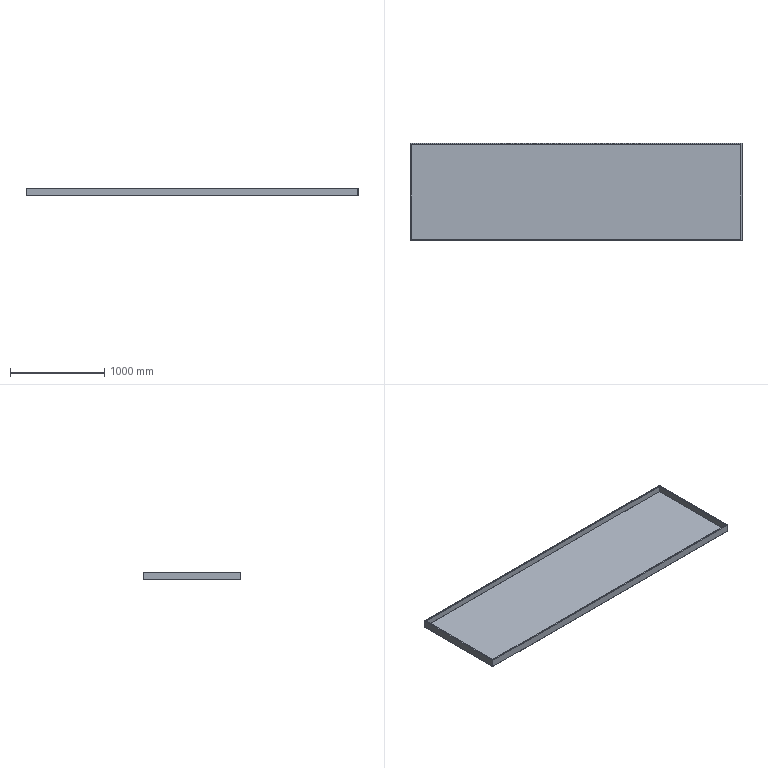Component | NX | DB2_21 | 1 solid | 16 faces | volume 6701262 mm3 | plane 16